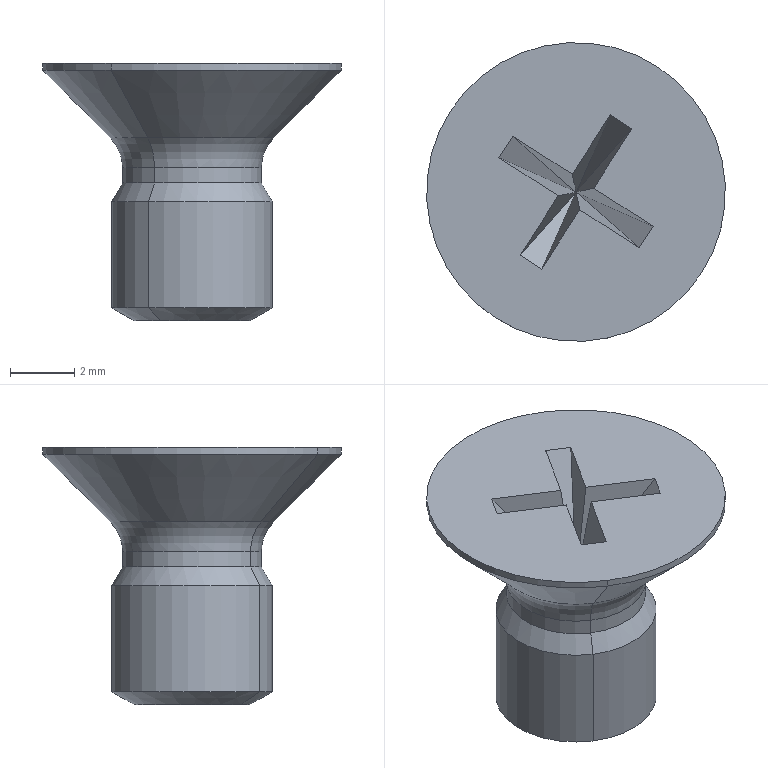Component | SolidWorks | MGL-PACK-03-00Fixture-1_PhillipsCountersunkScrewM5_8[GB_T819.1-2000]-1 | 1 solid | 28 faces | box 9.3 x 9.3 x 8 mm | volume 197 mm3 | plane 14 | cone 6 | cylinder 6 | torus 2 | commonest cylinder face diameters 5 x2 4.33 x2 9.3 x2
STEP:
#1=CARTESIAN_POINT('',(9.113,1.674,0.6496));
#2=VERTEX_POINT('',#1);
#3=CARTESIAN_POINT('',(9.036,1.554,0.6496));
#4=VERTEX_POINT('',#3);
#5=CARTESIAN_POINT('',(9.075,1.614,0.6496));
#6=DIRECTION('',(-0.,-0.,-1.));
#7=DIRECTION('',(0.5408,0.8411,0.));
#8=AXIS2_PLACEMENT_3D('',#5,#6,#7);
#9=CIRCLE('',#8,0.07115);
#10=EDGE_CURVE('',#2,#4,#9,.T.);
#11=ORIENTED_EDGE('',*,*,#10,.F.);
#12=CARTESIAN_POINT('',(9.128,1.697,0.6652));
#13=VERTEX_POINT('',#12);
#14=CARTESIAN_POINT('',(9.128,1.697,0.6652));
#15=DIRECTION('',(0.4696,0.7304,0.4959));
#16=VECTOR('',#15,39.37);
#17=LINE('',#14,#16);
#18=EDGE_CURVE('',#2,#13,#17,.T.);
#19=ORIENTED_EDGE('',*,*,#18,.T.);
#20=CARTESIAN_POINT('',(9.022,1.531,0.6652));
#21=VERTEX_POINT('',#20);
#22=CARTESIAN_POINT('',(9.075,1.614,0.6652));
#23=DIRECTION('',(-0.,-0.,-1.));
#24=DIRECTION('',(0.5408,0.8411,0.));
#25=AXIS2_PLACEMENT_3D('',#22,#23,#24);
#26=CIRCLE('',#25,0.09843);
#27=EDGE_CURVE('',#13,#21,#26,.T.);
#28=ORIENTED_EDGE('',*,*,#27,.T.);
#29=CARTESIAN_POINT('',(9.022,1.531,0.6652));
#30=DIRECTION('',(-0.4696,-0.7304,0.4959));
#31=VECTOR('',#30,39.37);
#32=LINE('',#29,#31);
#33=EDGE_CURVE('',#4,#21,#32,.T.);
#34=ORIENTED_EDGE('',*,*,#33,.F.);
#35=EDGE_LOOP('',(#11,#19,#28,#34));
#36=FACE_OUTER_BOUND('',#35,.T.);
#37=CARTESIAN_POINT('',(9.075,1.614,0.6652));
#38=DIRECTION('',(0.,0.,1.));
#39=DIRECTION('',(-0.5408,-0.8411,0.));
#40=AXIS2_PLACEMENT_3D('',#37,#38,#39);
#41=CONICAL_SURFACE('',#40,0.09843,1.052);
#42=ADVANCED_FACE('',(#36),#41,.T.);
#43=ORIENTED_EDGE('',*,*,#27,.F.);
#44=CARTESIAN_POINT('',(9.128,1.697,0.7953));
#45=VERTEX_POINT('',#44);
#46=CARTESIAN_POINT('',(9.128,1.697,0.9646));
#47=DIRECTION('',(0.,0.,1.));
#48=VECTOR('',#47,39.37);
#49=LINE('',#46,#48);
#50=EDGE_CURVE('',#13,#45,#49,.T.);
#51=ORIENTED_EDGE('',*,*,#50,.T.);
#52=CARTESIAN_POINT('',(9.022,1.531,0.7953));
#53=VERTEX_POINT('',#52);
#54=CARTESIAN_POINT('',(9.075,1.614,0.7953));
#55=DIRECTION('',(0.,0.,1.));
#56=DIRECTION('',(-0.5408,-0.8411,0.));
#57=AXIS2_PLACEMENT_3D('',#54,#55,#56);
#58=CIRCLE('',#57,0.09843);
#59=EDGE_CURVE('',#53,#45,#58,.T.);
#60=ORIENTED_EDGE('',*,*,#59,.F.);
#61=CARTESIAN_POINT('',(9.022,1.531,0.9646));
#62=DIRECTION('',(0.,0.,1.));
#63=VECTOR('',#62,39.37);
#64=LINE('',#61,#63);
#65=EDGE_CURVE('',#21,#53,#64,.T.);
#66=ORIENTED_EDGE('',*,*,#65,.F.);
#67=EDGE_LOOP('',(#43,#51,#60,#66));
#68=FACE_OUTER_BOUND('',#67,.T.);
#69=CARTESIAN_POINT('',(9.075,1.614,0.9646));
#70=DIRECTION('',(0.,0.,1.));
#71=DIRECTION('',(-0.5408,-0.8411,0.));
#72=AXIS2_PLACEMENT_3D('',#69,#70,#71);
#73=CYLINDRICAL_SURFACE('',#72,0.09843);
#74=ADVANCED_FACE('',(#68),#73,.T.);
#75=CARTESIAN_POINT('',(9.029,1.542,0.8181));
#76=VERTEX_POINT('',#75);
#77=CARTESIAN_POINT('',(9.121,1.686,0.8181));
#78=VERTEX_POINT('',#77);
#79=CARTESIAN_POINT('',(9.075,1.614,0.8181));
#80=DIRECTION('',(0.,0.,1.));
#81=DIRECTION('',(-0.5408,-0.8411,0.));
#82=AXIS2_PLACEMENT_3D('',#79,#80,#81);
#83=CIRCLE('',#82,0.08524);
#84=EDGE_CURVE('',#76,#78,#83,.T.);
#85=ORIENTED_EDGE('',*,*,#84,.F.);
#86=CARTESIAN_POINT('',(9.022,1.531,0.7953));
#87=DIRECTION('',(-0.2704,-0.4206,-0.866));
#88=VECTOR('',#87,39.37);
#89=LINE('',#86,#88);
#90=EDGE_CURVE('',#76,#53,#89,.T.);
#91=ORIENTED_EDGE('',*,*,#90,.T.);
#92=ORIENTED_EDGE('',*,*,#59,.T.);
#93=CARTESIAN_POINT('',(9.128,1.697,0.7953));
#94=DIRECTION('',(0.2704,0.4206,-0.866));
#95=VECTOR('',#94,39.37);
#96=LINE('',#93,#95);
#97=EDGE_CURVE('',#78,#45,#96,.T.);
#98=ORIENTED_EDGE('',*,*,#97,.F.);
#99=EDGE_LOOP('',(#85,#91,#92,#98));
#100=FACE_OUTER_BOUND('',#99,.T.);
#101=CARTESIAN_POINT('',(9.075,1.614,0.7953));
#102=DIRECTION('',(-0.,-0.,-1.));
#103=DIRECTION('',(0.5408,0.8411,0.));
#104=AXIS2_PLACEMENT_3D('',#101,#102,#103);
#105=CONICAL_SURFACE('',#104,0.09843,0.5236);
#106=ADVANCED_FACE('',(#100),#105,.T.);
#107=ORIENTED_EDGE('',*,*,#84,.T.);
#108=CARTESIAN_POINT('',(9.121,1.686,0.8371));
#109=VERTEX_POINT('',#108);
#110=CARTESIAN_POINT('',(9.121,1.686,0.9646));
#111=DIRECTION('',(0.,0.,1.));
#112=VECTOR('',#111,39.37);
#113=LINE('',#110,#112);
#114=EDGE_CURVE('',#78,#109,#113,.T.);
#115=ORIENTED_EDGE('',*,*,#114,.T.);
#116=CARTESIAN_POINT('',(9.029,1.542,0.8371));
#117=VERTEX_POINT('',#116);
#118=CARTESIAN_POINT('',(9.075,1.614,0.8371));
#119=DIRECTION('',(0.,0.,1.));
#120=DIRECTION('',(-0.5408,-0.8411,0.));
#121=AXIS2_PLACEMENT_3D('',#118,#119,#120);
#122=CIRCLE('',#121,0.08524);
#123=EDGE_CURVE('',#117,#109,#122,.T.);
#124=ORIENTED_EDGE('',*,*,#123,.F.);
#125=CARTESIAN_POINT('',(9.029,1.542,0.9646));
#126=DIRECTION('',(0.,0.,1.));
#127=VECTOR('',#126,39.37);
#128=LINE('',#125,#127);
#129=EDGE_CURVE('',#76,#117,#128,.T.);
#130=ORIENTED_EDGE('',*,*,#129,.F.);
#131=EDGE_LOOP('',(#107,#115,#124,#130));
#132=FACE_OUTER_BOUND('',#131,.T.);
#133=CARTESIAN_POINT('',(9.075,1.614,0.9646));
#134=DIRECTION('',(0.,0.,1.));
#135=DIRECTION('',(-0.5408,-0.8411,0.));
#136=AXIS2_PLACEMENT_3D('',#133,#134,#135);
#137=CYLINDRICAL_SURFACE('',#136,0.08524);
#138=ADVANCED_FACE('',(#132),#137,.T.);
#139=CARTESIAN_POINT('',(9.129,1.698,0.8733));
#140=VERTEX_POINT('',#139);
#141=CARTESIAN_POINT('',(9.021,1.53,0.8733));
#142=VERTEX_POINT('',#141);
#143=CARTESIAN_POINT('',(9.075,1.614,0.8733));
#144=DIRECTION('',(0.,0.,1.));
#145=DIRECTION('',(-0.5408,-0.8411,0.));
#146=AXIS2_PLACEMENT_3D('',#143,#144,#145);
#147=CIRCLE('',#146,0.1002);
#148=EDGE_CURVE('',#140,#142,#147,.T.);
#149=ORIENTED_EDGE('',*,*,#148,.F.);
#150=CARTESIAN_POINT('',(9.149,1.729,0.8371));
#151=DIRECTION('',(0.8411,-0.5408,0.));
#152=DIRECTION('',(0.5408,0.8411,0.));
#153=AXIS2_PLACEMENT_3D('',#150,#151,#152);
#154=CIRCLE('',#153,0.05118);
#155=EDGE_CURVE('',#140,#109,#154,.T.);
#156=ORIENTED_EDGE('',*,*,#155,.T.);
#157=CARTESIAN_POINT('',(9.075,1.614,0.8371));
#158=DIRECTION('',(0.,0.,1.));
#159=DIRECTION('',(-0.5408,-0.8411,0.));
#160=AXIS2_PLACEMENT_3D('',#157,#158,#159);
#161=CIRCLE('',#160,0.08524);
#162=EDGE_CURVE('',#109,#117,#161,.T.);
#163=ORIENTED_EDGE('',*,*,#162,.T.);
#164=CARTESIAN_POINT('',(9.001,1.499,0.8371));
#165=DIRECTION('',(-0.8411,0.5408,-0.));
#166=DIRECTION('',(-0.5408,-0.8411,0.));
#167=AXIS2_PLACEMENT_3D('',#164,#165,#166);
#168=CIRCLE('',#167,0.05118);
#169=EDGE_CURVE('',#142,#117,#168,.T.);
#170=ORIENTED_EDGE('',*,*,#169,.F.);
#171=EDGE_LOOP('',(#149,#156,#163,#170));
#172=FACE_OUTER_BOUND('',#171,.T.);
#173=CARTESIAN_POINT('',(9.075,1.614,0.8371));
#174=DIRECTION('',(0.,0.,1.));
#175=DIRECTION('',(-0.5408,-0.8411,0.));
#176=AXIS2_PLACEMENT_3D('',#173,#174,#175);
#177=TOROIDAL_SURFACE('',#176,0.1364,0.05118);
#178=ADVANCED_FACE('',(#172),#177,.F.);
#179=CARTESIAN_POINT('',(9.075,1.614,0.8733));
#180=DIRECTION('',(0.,0.,1.));
#181=DIRECTION('',(-0.5408,-0.8411,0.));
#182=AXIS2_PLACEMENT_3D('',#179,#180,#181);
#183=CIRCLE('',#182,0.1002);
#184=EDGE_CURVE('',#142,#140,#183,.T.);
#185=ORIENTED_EDGE('',*,*,#184,.T.);
#186=CARTESIAN_POINT('',(9.174,1.768,0.9561));
#187=VERTEX_POINT('',#186);
#188=CARTESIAN_POINT('',(9.129,1.698,0.8733));
#189=DIRECTION('',(0.3824,0.5948,0.7071));
#190=VECTOR('',#189,39.37);
#191=LINE('',#188,#190);
#192=EDGE_CURVE('',#140,#187,#191,.T.);
#193=ORIENTED_EDGE('',*,*,#192,.T.);
#194=CARTESIAN_POINT('',(8.976,1.46,0.9561));
#195=VERTEX_POINT('',#194);
#196=CARTESIAN_POINT('',(9.075,1.614,0.9561));
#197=DIRECTION('',(0.,0.,1.));
#198=DIRECTION('',(-0.5408,-0.8411,0.));
#199=AXIS2_PLACEMENT_3D('',#196,#197,#198);
#200=CIRCLE('',#199,0.1831);
#201=EDGE_CURVE('',#195,#187,#200,.T.);
#202=ORIENTED_EDGE('',*,*,#201,.F.);
#203=CARTESIAN_POINT('',(9.021,1.53,0.8733));
#204=DIRECTION('',(-0.3824,-0.5948,0.7071));
#205=VECTOR('',#204,39.37);
#206=LINE('',#203,#205);
#207=EDGE_CURVE('',#142,#195,#206,.T.);
#208=ORIENTED_EDGE('',*,*,#207,.F.);
#209=EDGE_LOOP('',(#185,#193,#202,#208));
#210=FACE_OUTER_BOUND('',#209,.T.);
#211=CARTESIAN_POINT('',(9.075,1.614,0.8733));
#212=DIRECTION('',(0.,0.,1.));
#213=DIRECTION('',(-0.5408,-0.8411,0.));
#214=AXIS2_PLACEMENT_3D('',#211,#212,#213);
#215=CONICAL_SURFACE('',#214,0.1002,0.7854);
#216=ADVANCED_FACE('',(#210),#215,.T.);
#217=ORIENTED_EDGE('',*,*,#201,.T.);
#218=CARTESIAN_POINT('',(9.174,1.768,0.9646));
#219=VERTEX_POINT('',#218);
#220=CARTESIAN_POINT('',(9.174,1.768,0.9646));
#221=DIRECTION('',(0.,0.,1.));
#222=VECTOR('',#221,39.37);
#223=LINE('',#220,#222);
#224=EDGE_CURVE('',#187,#219,#223,.T.);
#225=ORIENTED_EDGE('',*,*,#224,.T.);
#226=CARTESIAN_POINT('',(8.976,1.46,0.9646));
#227=VERTEX_POINT('',#226);
#228=CARTESIAN_POINT('',(9.075,1.614,0.9646));
#229=DIRECTION('',(0.,0.,1.));
#230=DIRECTION('',(-0.5408,-0.8411,0.));
#231=AXIS2_PLACEMENT_3D('',#228,#229,#230);
#232=CIRCLE('',#231,0.1831);
#233=EDGE_CURVE('',#227,#219,#232,.T.);
#234=ORIENTED_EDGE('',*,*,#233,.F.);
#235=CARTESIAN_POINT('',(8.976,1.46,0.9646));
#236=DIRECTION('',(0.,0.,1.));
#237=VECTOR('',#236,39.37);
#238=LINE('',#235,#237);
#239=EDGE_CURVE('',#195,#227,#238,.T.);
#240=ORIENTED_EDGE('',*,*,#239,.F.);
#241=EDGE_LOOP('',(#217,#225,#234,#240));
#242=FACE_OUTER_BOUND('',#241,.T.);
#243=CARTESIAN_POINT('',(9.075,1.614,0.9646));
#244=DIRECTION('',(0.,0.,1.));
#245=DIRECTION('',(-0.5408,-0.8411,0.));
#246=AXIS2_PLACEMENT_3D('',#243,#244,#245);
#247=CYLINDRICAL_SURFACE('',#246,0.1831);
#248=ADVANCED_FACE('',(#242),#247,.T.);
#249=ORIENTED_EDGE('',*,*,#233,.T.);
#250=CARTESIAN_POINT('',(9.075,1.614,0.9646));
#251=DIRECTION('',(0.,0.,1.));
#252=DIRECTION('',(-0.5408,-0.8411,0.));
#253=AXIS2_PLACEMENT_3D('',#250,#251,#252);
#254=CIRCLE('',#253,0.1831);
#255=EDGE_CURVE('',#219,#227,#254,.T.);
#256=ORIENTED_EDGE('',*,*,#255,.T.);
#257=EDGE_LOOP('',(#249,#256));
#258=FACE_OUTER_BOUND('',#257,.T.);
#259=CARTESIAN_POINT('',(9.08,1.592,0.9646));
#260=VERTEX_POINT('',#259);
#261=CARTESIAN_POINT('',(9.152,1.546,0.9646));
#262=VERTEX_POINT('',#261);
#263=CARTESIAN_POINT('',(9.152,1.546,0.9646));
#264=DIRECTION('',(0.8411,-0.5408,0.));
#265=VECTOR('',#264,39.37);
#266=LINE('',#263,#265);
#267=EDGE_CURVE('',#260,#262,#266,.T.);
#268=ORIENTED_EDGE('',*,*,#267,.F.);
#269=CARTESIAN_POINT('',(9.033,1.52,0.9646));
#270=VERTEX_POINT('',#269);
#271=CARTESIAN_POINT('',(9.143,1.692,0.9646));
#272=DIRECTION('',(0.5408,0.8411,-0.));
#273=VECTOR('',#272,39.37);
#274=LINE('',#271,#273);
#275=EDGE_CURVE('',#270,#260,#274,.T.);
#276=ORIENTED_EDGE('',*,*,#275,.F.);
#277=CARTESIAN_POINT('',(9.006,1.537,0.9646));
#278=VERTEX_POINT('',#277);
#279=CARTESIAN_POINT('',(9.033,1.52,0.9646));
#280=DIRECTION('',(0.8411,-0.5408,0.));
#281=VECTOR('',#280,39.37);
#282=LINE('',#279,#281);
#283=EDGE_CURVE('',#278,#270,#282,.T.);
#284=ORIENTED_EDGE('',*,*,#283,.F.);
#285=CARTESIAN_POINT('',(9.053,1.609,0.9646));
#286=VERTEX_POINT('',#285);
#287=CARTESIAN_POINT('',(9.117,1.709,0.9646));
#288=DIRECTION('',(-0.5408,-0.8411,0.));
#289=VECTOR('',#288,39.37);
#290=LINE('',#287,#289);
#291=EDGE_CURVE('',#286,#278,#290,.T.);
#292=ORIENTED_EDGE('',*,*,#291,.F.);
#293=CARTESIAN_POINT('',(8.98,1.656,0.9646));
#294=VERTEX_POINT('',#293);
#295=CARTESIAN_POINT('',(9.152,1.546,0.9646));
#296=DIRECTION('',(0.8411,-0.5408,0.));
#297=VECTOR('',#296,39.37);
#298=LINE('',#295,#297);
#299=EDGE_CURVE('',#294,#286,#298,.T.);
#300=ORIENTED_EDGE('',*,*,#299,.F.);
#301=CARTESIAN_POINT('',(8.997,1.683,0.9646));
#302=VERTEX_POINT('',#301);
#303=CARTESIAN_POINT('',(8.98,1.656,0.9646));
#304=DIRECTION('',(-0.5408,-0.8411,0.));
#305=VECTOR('',#304,39.37);
#306=LINE('',#303,#305);
#307=EDGE_CURVE('',#302,#294,#306,.T.);
#308=ORIENTED_EDGE('',*,*,#307,.F.);
#309=CARTESIAN_POINT('',(9.07,1.636,0.9646));
#310=VERTEX_POINT('',#309);
#311=CARTESIAN_POINT('',(9.169,1.572,0.9646));
#312=DIRECTION('',(-0.8411,0.5408,-0.));
#313=VECTOR('',#312,39.37);
#314=LINE('',#311,#313);
#315=EDGE_CURVE('',#310,#302,#314,.T.);
#316=ORIENTED_EDGE('',*,*,#315,.F.);
#317=CARTESIAN_POINT('',(9.117,1.709,0.9646));
#318=VERTEX_POINT('',#317);
#319=CARTESIAN_POINT('',(9.117,1.709,0.9646));
#320=DIRECTION('',(-0.5408,-0.8411,0.));
#321=VECTOR('',#320,39.37);
#322=LINE('',#319,#321);
#323=EDGE_CURVE('',#318,#310,#322,.T.);
#324=ORIENTED_EDGE('',*,*,#323,.F.);
#325=CARTESIAN_POINT('',(9.143,1.692,0.9646));
#326=VERTEX_POINT('',#325);
#327=CARTESIAN_POINT('',(9.143,1.692,0.9646));
#328=DIRECTION('',(-0.8411,0.5408,-0.));
#329=VECTOR('',#328,39.37);
#330=LINE('',#327,#329);
#331=EDGE_CURVE('',#326,#318,#330,.T.);
#332=ORIENTED_EDGE('',*,*,#331,.F.);
#333=CARTESIAN_POINT('',(9.097,1.619,0.9646));
#334=VERTEX_POINT('',#333);
#335=CARTESIAN_POINT('',(9.143,1.692,0.9646));
#336=DIRECTION('',(0.5408,0.8411,-0.));
#337=VECTOR('',#336,39.37);
#338=LINE('',#335,#337);
#339=EDGE_CURVE('',#334,#326,#338,.T.);
#340=ORIENTED_EDGE('',*,*,#339,.F.);
#341=CARTESIAN_POINT('',(9.169,1.572,0.9646));
#342=VERTEX_POINT('',#341);
#343=CARTESIAN_POINT('',(9.169,1.572,0.9646));
#344=DIRECTION('',(-0.8411,0.5408,-0.));
#345=VECTOR('',#344,39.37);
#346=LINE('',#343,#345);
#347=EDGE_CURVE('',#342,#334,#346,.T.);
#348=ORIENTED_EDGE('',*,*,#347,.F.);
#349=CARTESIAN_POINT('',(9.152,1.546,0.9646));
#350=DIRECTION('',(0.5408,0.8411,-0.));
#351=VECTOR('',#350,39.37);
#352=LINE('',#349,#351);
#353=EDGE_CURVE('',#262,#342,#352,.T.);
#354=ORIENTED_EDGE('',*,*,#353,.F.);
#355=EDGE_LOOP('',(#268,#276,#284,#292,#300,#308,#316,#324,#332,#340,#348,#354));
#356=FACE_BOUND('',#355,.T.);
#357=CARTESIAN_POINT('',(9.075,1.614,0.9646));
#358=DIRECTION('',(-0.,-0.,-1.));
#359=DIRECTION('',(0.5408,0.8411,-0.));
#360=AXIS2_PLACEMENT_3D('',#357,#358,#359);
#361=PLANE('',#360);
#362=ADVANCED_FACE('',(#258,#356),#361,.F.);
#363=ORIENTED_EDGE('',*,*,#275,.T.);
#364=CARTESIAN_POINT('',(9.075,1.614,0.8386));
#365=VERTEX_POINT('',#364);
#366=CARTESIAN_POINT('',(9.075,1.614,0.8386));
#367=DIRECTION('',(-0.03697,0.1701,-0.9847));
#368=VECTOR('',#367,39.37);
#369=LINE('',#366,#368);
#370=EDGE_CURVE('',#260,#365,#369,.T.);
#371=ORIENTED_EDGE('',*,*,#370,.T.);
#372=CARTESIAN_POINT('',(9.033,1.52,0.9646));
#373=DIRECTION('',(0.2582,0.5802,-0.7725));
#374=VECTOR('',#373,39.37);
#375=LINE('',#372,#374);
#376=EDGE_CURVE('',#270,#365,#375,.T.);
#377=ORIENTED_EDGE('',*,*,#376,.F.);
#378=EDGE_LOOP('',(#363,#371,#377));
#379=FACE_OUTER_BOUND('',#378,.T.);
#380=CARTESIAN_POINT('',(9.075,1.614,0.8386));
#381=DIRECTION('',(-0.8347,0.5366,0.124));
#382=DIRECTION('',(-0.1043,0.06708,-0.9923));
#383=AXIS2_PLACEMENT_3D('',#380,#381,#382);
#384=PLANE('',#383);
#385=ADVANCED_FACE('',(#379),#384,.T.);
#386=CARTESIAN_POINT('',(9.143,1.692,0.9646));
#387=DIRECTION('',(-0.4207,-0.4757,-0.7725));
#388=VECTOR('',#387,39.37);
#389=LINE('',#386,#388);
#390=EDGE_CURVE('',#326,#365,#389,.T.);
#391=ORIENTED_EDGE('',*,*,#390,.T.);
#392=CARTESIAN_POINT('',(9.075,1.614,0.8386));
#393=DIRECTION('',(0.1701,0.03697,0.9847));
#394=VECTOR('',#393,39.37);
#395=LINE('',#392,#394);
#396=EDGE_CURVE('',#365,#334,#395,.T.);
#397=ORIENTED_EDGE('',*,*,#396,.T.);
#398=ORIENTED_EDGE('',*,*,#339,.T.);
#399=EDGE_LOOP('',(#391,#397,#398));
#400=FACE_OUTER_BOUND('',#399,.T.);
#401=CARTESIAN_POINT('',(9.075,1.614,0.8386));
#402=DIRECTION('',(-0.8347,0.5366,0.124));
#403=DIRECTION('',(-0.1043,0.06708,-0.9923));
#404=AXIS2_PLACEMENT_3D('',#401,#402,#403);
#405=PLANE('',#404);
#406=ADVANCED_FACE('',(#400),#405,.T.);
#407=CARTESIAN_POINT('',(9.006,1.537,0.9646));
#408=DIRECTION('',(0.4207,0.4757,-0.7725));
#409=VECTOR('',#408,39.37);
#410=LINE('',#407,#409);
#411=EDGE_CURVE('',#278,#365,#410,.T.);
#412=ORIENTED_EDGE('',*,*,#411,.T.);
#413=CARTESIAN_POINT('',(9.075,1.614,0.8386));
#414=DIRECTION('',(-0.1701,-0.03697,0.9847));
#415=VECTOR('',#414,39.37);
#416=LINE('',#413,#415);
#417=EDGE_CURVE('',#365,#286,#416,.T.);
#418=ORIENTED_EDGE('',*,*,#417,.T.);
#419=ORIENTED_EDGE('',*,*,#291,.T.);
#420=EDGE_LOOP('',(#412,#418,#419));
#421=FACE_OUTER_BOUND('',#420,.T.);
#422=CARTESIAN_POINT('',(9.075,1.614,0.8386));
#423=DIRECTION('',(0.8347,-0.5366,0.124));
#424=DIRECTION('',(-0.1043,0.06708,0.9923));
#425=AXIS2_PLACEMENT_3D('',#422,#423,#424);
#426=PLANE('',#425);
#427=ADVANCED_FACE('',(#421),#426,.T.);
#428=ORIENTED_EDGE('',*,*,#323,.T.);
#429=CARTESIAN_POINT('',(9.075,1.614,0.8386));
#430=DIRECTION('',(0.03697,-0.1701,-0.9847));
#431=VECTOR('',#430,39.37);
#432=LINE('',#429,#431);
#433=EDGE_CURVE('',#310,#365,#432,.T.);
#434=ORIENTED_EDGE('',*,*,#433,.T.);
#435=CARTESIAN_POINT('',(9.117,1.709,0.9646));
#436=DIRECTION('',(-0.2582,-0.5802,-0.7725));
#437=VECTOR('',#436,39.37);
#438=LINE('',#435,#437);
#439=EDGE_CURVE('',#318,#365,#438,.T.);
#440=ORIENTED_EDGE('',*,*,#439,.F.);
#441=EDGE_LOOP('',(#428,#434,#440));
#442=FACE_OUTER_BOUND('',#441,.T.);
#443=CARTESIAN_POINT('',(9.075,1.614,0.8386));
#444=DIRECTION('',(0.8347,-0.5366,0.124));
#445=DIRECTION('',(-0.1043,0.06708,0.9923));
#446=AXIS2_PLACEMENT_3D('',#443,#444,#445);
#447=PLANE('',#446);
#448=ADVANCED_FACE('',(#442),#447,.T.);
#449=ORIENTED_EDGE('',*,*,#224,.F.);
#450=CARTESIAN_POINT('',(9.075,1.614,0.9561));
#451=DIRECTION('',(0.,0.,1.));
#452=DIRECTION('',(-0.5408,-0.8411,0.));
#453=AXIS2_PLACEMENT_3D('',#450,#451,#452);
#454=CIRCLE('',#453,0.1831);
#455=EDGE_CURVE('',#187,#195,#454,.T.);
#456=ORIENTED_EDGE('',*,*,#455,.T.);
#457=ORIENTED_EDGE('',*,*,#239,.T.);
#458=ORIENTED_EDGE('',*,*,#255,.F.);
#459=EDGE_LOOP('',(#449,#456,#457,#458));
#460=FACE_OUTER_BOUND('',#459,.T.);
#461=CARTESIAN_POINT('',(9.075,1.614,0.9646));
#462=DIRECTION('',(0.,0.,1.));
#463=DIRECTION('',(-0.5408,-0.8411,0.));
#464=AXIS2_PLACEMENT_3D('',#461,#462,#463);
#465=CYLINDRICAL_SURFACE('',#464,0.1831);
#466=ADVANCED_FACE('',(#460),#465,.T.);
#467=ORIENTED_EDGE('',*,*,#192,.F.);
#468=ORIENTED_EDGE('',*,*,#148,.T.);
#469=ORIENTED_EDGE('',*,*,#207,.T.);
#470=ORIENTED_EDGE('',*,*,#455,.F.);
#471=EDGE_LOOP('',(#467,#468,#469,#470));
#472=FACE_OUTER_BOUND('',#471,.T.);
#473=CARTESIAN_POINT('',(9.075,1.614,0.8733));
#474=DIRECTION('',(0.,0.,1.));
#475=DIRECTION('',(-0.5408,-0.8411,0.));
#476=AXIS2_PLACEMENT_3D('',#473,#474,#475);
#477=CONICAL_SURFACE('',#476,0.1002,0.7854);
#478=ADVANCED_FACE('',(#472),#477,.T.);
#479=ORIENTED_EDGE('',*,*,#155,.F.);
#480=ORIENTED_EDGE('',*,*,#184,.F.);
#481=ORIENTED_EDGE('',*,*,#169,.T.);
#482=ORIENTED_EDGE('',*,*,#123,.T.);
#483=EDGE_LOOP('',(#479,#480,#481,#482));
#484=FACE_OUTER_BOUND('',#483,.T.);
#485=CARTESIAN_POINT('',(9.075,1.614,0.8371));
#486=DIRECTION('',(0.,0.,1.));
#487=DIRECTION('',(-0.5408,-0.8411,0.));
#488=AXIS2_PLACEMENT_3D('',#485,#486,#487);
#489=TOROIDAL_SURFACE('',#488,0.1364,0.05118);
#490=ADVANCED_FACE('',(#484),#489,.F.);
#491=ORIENTED_EDGE('',*,*,#114,.F.);
#492=CARTESIAN_POINT('',(9.075,1.614,0.8181));
#493=DIRECTION('',(0.,0.,1.));
#494=DIRECTION('',(-0.5408,-0.8411,0.));
#495=AXIS2_PLACEMENT_3D('',#492,#493,#494);
#496=CIRCLE('',#495,0.08524);
#497=EDGE_CURVE('',#78,#76,#496,.T.);
#498=ORIENTED_EDGE('',*,*,#497,.T.);
#499=ORIENTED_EDGE('',*,*,#129,.T.);
#500=ORIENTED_EDGE('',*,*,#162,.F.);
#501=EDGE_LOOP('',(#491,#498,#499,#500));
#502=FACE_OUTER_BOUND('',#501,.T.);
#503=CARTESIAN_POINT('',(9.075,1.614,0.9646));
#504=DIRECTION('',(0.,0.,1.));
#505=DIRECTION('',(-0.5408,-0.8411,0.));
#506=AXIS2_PLACEMENT_3D('',#503,#504,#505);
#507=CYLINDRICAL_SURFACE('',#506,0.08524);
#508=ADVANCED_FACE('',(#502),#507,.T.);
#509=ORIENTED_EDGE('',*,*,#90,.F.);
#510=ORIENTED_EDGE('',*,*,#497,.F.);
#511=ORIENTED_EDGE('',*,*,#97,.T.);
#512=CARTESIAN_POINT('',(9.075,1.614,0.7953));
#513=DIRECTION('',(0.,0.,1.));
#514=DIRECTION('',(-0.5408,-0.8411,0.));
#515=AXIS2_PLACEMENT_3D('',#512,#513,#514);
#516=CIRCLE('',#515,0.09843);
#517=EDGE_CURVE('',#45,#53,#516,.T.);
#518=ORIENTED_EDGE('',*,*,#517,.T.);
#519=EDGE_LOOP('',(#509,#510,#511,#518));
#520=FACE_OUTER_BOUND('',#519,.T.);
#521=CARTESIAN_POINT('',(9.075,1.614,0.7953));
#522=DIRECTION('',(-0.,-0.,-1.));
#523=DIRECTION('',(0.5408,0.8411,0.));
#524=AXIS2_PLACEMENT_3D('',#521,#522,#523);
#525=CONICAL_SURFACE('',#524,0.09843,0.5236);
#526=ADVANCED_FACE('',(#520),#525,.T.);
#527=ORIENTED_EDGE('',*,*,#50,.F.);
#528=CARTESIAN_POINT('',(9.075,1.614,0.6652));
#529=DIRECTION('',(-0.,-0.,-1.));
#530=DIRECTION('',(0.5408,0.8411,0.));
#531=AXIS2_PLACEMENT_3D('',#528,#529,#530);
#532=CIRCLE('',#531,0.09843);
#533=EDGE_CURVE('',#21,#13,#532,.T.);
#534=ORIENTED_EDGE('',*,*,#533,.F.);
#535=ORIENTED_EDGE('',*,*,#65,.T.);
#536=ORIENTED_EDGE('',*,*,#517,.F.);
#537=EDGE_LOOP('',(#527,#534,#535,#536));
#538=FACE_OUTER_BOUND('',#537,.T.);
#539=CARTESIAN_POINT('',(9.075,1.614,0.9646));
#540=DIRECTION('',(0.,0.,1.));
#541=DIRECTION('',(-0.5408,-0.8411,0.));
#542=AXIS2_PLACEMENT_3D('',#539,#540,#541);
#543=CYLINDRICAL_SURFACE('',#542,0.09843);
#544=ADVANCED_FACE('',(#538),#543,.T.);
#545=ORIENTED_EDGE('',*,*,#18,.F.);
#546=CARTESIAN_POINT('',(9.075,1.614,0.6496));
#547=DIRECTION('',(-0.,-0.,-1.));
#548=DIRECTION('',(0.5408,0.8411,0.));
#549=AXIS2_PLACEMENT_3D('',#546,#547,#548);
#550=CIRCLE('',#549,0.07115);
#551=EDGE_CURVE('',#4,#2,#550,.T.);
#552=ORIENTED_EDGE('',*,*,#551,.F.);
#553=ORIENTED_EDGE('',*,*,#33,.T.);
#554=ORIENTED_EDGE('',*,*,#533,.T.);
#555=EDGE_LOOP('',(#545,#552,#553,#554));
#556=FACE_OUTER_BOUND('',#555,.T.);
#557=CARTESIAN_POINT('',(9.075,1.614,0.6652));
#558=DIRECTION('',(0.,0.,1.));
#559=DIRECTION('',(-0.5408,-0.8411,0.));
#560=AXIS2_PLACEMENT_3D('',#557,#558,#559);
#561=CONICAL_SURFACE('',#560,0.09843,1.052);
#562=ADVANCED_FACE('',(#556),#561,.T.);
#563=ORIENTED_EDGE('',*,*,#551,.T.);
#564=ORIENTED_EDGE('',*,*,#10,.T.);
#565=EDGE_LOOP('',(#563,#564));
#566=FACE_OUTER_BOUND('',#565,.T.);
#567=CARTESIAN_POINT('',(9.158,1.561,0.6496));
#568=DIRECTION('',(0.,0.,1.));
#569=DIRECTION('',(-0.5408,-0.8411,0.));
#570=AXIS2_PLACEMENT_3D('',#567,#568,#569);
#571=PLANE('',#570);
#572=ADVANCED_FACE('',(#566),#571,.F.);
#573=ORIENTED_EDGE('',*,*,#390,.F.);
#574=ORIENTED_EDGE('',*,*,#331,.T.);
#575=ORIENTED_EDGE('',*,*,#439,.T.);
#576=EDGE_LOOP('',(#573,#574,#575));
#577=FACE_OUTER_BOUND('',#576,.T.);
#578=CARTESIAN_POINT('',(9.143,1.692,0.9646));
#579=DIRECTION('',(0.4197,0.6528,-0.6306));
#580=DIRECTION('',(0.341,0.5304,0.7761));
#581=AXIS2_PLACEMENT_3D('',#578,#579,#580);
#582=PLANE('',#581);
#583=ADVANCED_FACE('',(#577),#582,.F.);
#584=ORIENTED_EDGE('',*,*,#411,.F.);
#585=ORIENTED_EDGE('',*,*,#283,.T.);
#586=ORIENTED_EDGE('',*,*,#376,.T.);
#587=EDGE_LOOP('',(#584,#585,#586));
#588=FACE_OUTER_BOUND('',#587,.T.);
#589=CARTESIAN_POINT('',(9.006,1.537,0.9646));
#590=DIRECTION('',(-0.4197,-0.6528,-0.6306));
#591=DIRECTION('',(0.341,0.5304,-0.7761));
#592=AXIS2_PLACEMENT_3D('',#589,#590,#591);
#593=PLANE('',#592);
#594=ADVANCED_FACE('',(#588),#593,.F.);
#595=CARTESIAN_POINT('',(8.98,1.656,0.9646));
#596=DIRECTION('',(0.5802,-0.2582,-0.7725));
#597=VECTOR('',#596,39.37);
#598=LINE('',#595,#597);
#599=EDGE_CURVE('',#294,#365,#598,.T.);
#600=ORIENTED_EDGE('',*,*,#599,.F.);
#601=ORIENTED_EDGE('',*,*,#299,.T.);
#602=ORIENTED_EDGE('',*,*,#417,.F.);
#603=EDGE_LOOP('',(#600,#601,#602));
#604=FACE_OUTER_BOUND('',#603,.T.);
#605=CARTESIAN_POINT('',(9.075,1.614,0.8386));
#606=DIRECTION('',(0.5366,0.8347,0.124));
#607=DIRECTION('',(0.06708,0.1043,-0.9923));
#608=AXIS2_PLACEMENT_3D('',#605,#606,#607);
#609=PLANE('',#608);
#610=ADVANCED_FACE('',(#604),#609,.T.);
#611=ORIENTED_EDGE('',*,*,#315,.T.);
#612=CARTESIAN_POINT('',(8.997,1.683,0.9646));
#613=DIRECTION('',(0.4757,-0.4207,-0.7725));
#614=VECTOR('',#613,39.37);
#615=LINE('',#612,#614);
#616=EDGE_CURVE('',#302,#365,#615,.T.);
#617=ORIENTED_EDGE('',*,*,#616,.T.);
#618=ORIENTED_EDGE('',*,*,#433,.F.);
#619=EDGE_LOOP('',(#611,#617,#618));
#620=FACE_OUTER_BOUND('',#619,.T.);
#621=CARTESIAN_POINT('',(9.075,1.614,0.8386));
#622=DIRECTION('',(-0.5366,-0.8347,0.124));
#623=DIRECTION('',(0.06708,0.1043,0.9923));
#624=AXIS2_PLACEMENT_3D('',#621,#622,#623);
#625=PLANE('',#624);
#626=ADVANCED_FACE('',(#620),#625,.T.);
#627=ORIENTED_EDGE('',*,*,#616,.F.);
#628=ORIENTED_EDGE('',*,*,#307,.T.);
#629=ORIENTED_EDGE('',*,*,#599,.T.);
#630=EDGE_LOOP('',(#627,#628,#629));
#631=FACE_OUTER_BOUND('',#630,.T.);
#632=CARTESIAN_POINT('',(8.997,1.683,0.9646));
#633=DIRECTION('',(-0.6528,0.4197,-0.6306));
#634=DIRECTION('',(0.5304,-0.341,-0.7761));
#635=AXIS2_PLACEMENT_3D('',#632,#633,#634);
#636=PLANE('',#635);
#637=ADVANCED_FACE('',(#631),#636,.F.);
#638=ORIENTED_EDGE('',*,*,#267,.T.);
#639=CARTESIAN_POINT('',(9.152,1.546,0.9646));
#640=DIRECTION('',(-0.4757,0.4207,-0.7725));
#641=VECTOR('',#640,39.37);
#642=LINE('',#639,#641);
#643=EDGE_CURVE('',#262,#365,#642,.T.);
#644=ORIENTED_EDGE('',*,*,#643,.T.);
#645=ORIENTED_EDGE('',*,*,#370,.F.);
#646=EDGE_LOOP('',(#638,#644,#645));
#647=FACE_OUTER_BOUND('',#646,.T.);
#648=CARTESIAN_POINT('',(9.075,1.614,0.8386));
#649=DIRECTION('',(0.5366,0.8347,0.124));
#650=DIRECTION('',(0.06708,0.1043,-0.9923));
#651=AXIS2_PLACEMENT_3D('',#648,#649,#650);
#652=PLANE('',#651);
#653=ADVANCED_FACE('',(#647),#652,.T.);
#654=CARTESIAN_POINT('',(9.169,1.572,0.9646));
#655=DIRECTION('',(-0.5802,0.2582,-0.7725));
#656=VECTOR('',#655,39.37);
#657=LINE('',#654,#656);
#658=EDGE_CURVE('',#342,#365,#657,.T.);
#659=ORIENTED_EDGE('',*,*,#658,.F.);
#660=ORIENTED_EDGE('',*,*,#347,.T.);
#661=ORIENTED_EDGE('',*,*,#396,.F.);
#662=EDGE_LOOP('',(#659,#660,#661));
#663=FACE_OUTER_BOUND('',#662,.T.);
#664=CARTESIAN_POINT('',(9.075,1.614,0.8386));
#665=DIRECTION('',(-0.5366,-0.8347,0.124));
#666=DIRECTION('',(0.06708,0.1043,0.9923));
#667=AXIS2_PLACEMENT_3D('',#664,#665,#666);
#668=PLANE('',#667);
#669=ADVANCED_FACE('',(#663),#668,.T.);
#670=ORIENTED_EDGE('',*,*,#643,.F.);
#671=ORIENTED_EDGE('',*,*,#353,.T.);
#672=ORIENTED_EDGE('',*,*,#658,.T.);
#673=EDGE_LOOP('',(#670,#671,#672));
#674=FACE_OUTER_BOUND('',#673,.T.);
#675=CARTESIAN_POINT('',(9.152,1.546,0.9646));
#676=DIRECTION('',(0.6528,-0.4197,-0.6306));
#677=DIRECTION('',(0.5304,-0.341,0.7761));
#678=AXIS2_PLACEMENT_3D('',#675,#676,#677);
#679=PLANE('',#678);
#680=ADVANCED_FACE('',(#674),#679,.F.);
#681=CLOSED_SHELL('',(#42,#74,#106,#138,#178,#216,#248,#362,#385,#406,#427,#448,#466,#478,#490,#508,#526,#544,#562,#572,#583,#594,#610,#626,#637,#653,#669,#680));
#682=MANIFOLD_SOLID_BREP('',#681);
#683=CARTESIAN_POINT('',(0.,0.,0.));
#684=DIRECTION('',(0.,0.,1.));
#685=DIRECTION('',(1.,0.,0.));
#686=AXIS2_PLACEMENT_3D('',#683,#684,#685);
#687=(LENGTH_UNIT()NAMED_UNIT(*)SI_UNIT($,.METRE.));
#688=LENGTH_MEASURE_WITH_UNIT(LENGTH_MEASURE(0.0254),#687);
#689=DIMENSIONAL_EXPONENTS(1.,0.,0.,0.,0.,0.,0.);
#690=(CONVERSION_BASED_UNIT('',#688)LENGTH_UNIT()NAMED_UNIT(#689));
#691=UNCERTAINTY_MEASURE_WITH_UNIT(LENGTH_MEASURE(0.00001),#690,'','');
#692=(NAMED_UNIT(*)PLANE_ANGLE_UNIT()SI_UNIT($,.RADIAN.));
#693=(NAMED_UNIT(*)SI_UNIT($,.STERADIAN.)SOLID_ANGLE_UNIT());
#694=(GEOMETRIC_REPRESENTATION_CONTEXT(3)GLOBAL_UNCERTAINTY_ASSIGNED_CONTEXT((#691))GLOBAL_UNIT_ASSIGNED_CONTEXT((#690,#692,#693))REPRESENTATION_CONTEXT('',''));
#695=ADVANCED_BREP_SHAPE_REPRESENTATION('',(#682,#686),#694);
#696=COLOUR_RGB('',0.7922,0.8196,0.9333);
#697=FILL_AREA_STYLE_COLOUR('',#696);
#698=FILL_AREA_STYLE('',(#697));
#699=SURFACE_STYLE_FILL_AREA(#698);
#700=SURFACE_SIDE_STYLE('',(#699));
#701=SURFACE_STYLE_USAGE(.BOTH.,#700);
#702=PRESENTATION_STYLE_ASSIGNMENT((#701));
#703=STYLED_ITEM('',(#702),#682);
#704=PRESENTATION_LAYER_ASSIGNMENT('','',(#703));
#705=(LENGTH_UNIT()NAMED_UNIT(*)SI_UNIT($,.METRE.));
#706=LENGTH_MEASURE_WITH_UNIT(LENGTH_MEASURE(0.0254),#705);
#707=DIMENSIONAL_EXPONENTS(1.,0.,0.,0.,0.,0.,0.);
#708=(CONVERSION_BASED_UNIT('',#706)LENGTH_UNIT()NAMED_UNIT(#707));
#709=UNCERTAINTY_MEASURE_WITH_UNIT(LENGTH_MEASURE(0.00001),#708,'','');
#710=(NAMED_UNIT(*)PLANE_ANGLE_UNIT()SI_UNIT($,.RADIAN.));
#711=(NAMED_UNIT(*)SI_UNIT($,.STERADIAN.)SOLID_ANGLE_UNIT());
#712=(GEOMETRIC_REPRESENTATION_CONTEXT(3)GLOBAL_UNCERTAINTY_ASSIGNED_CONTEXT((#709))GLOBAL_UNIT_ASSIGNED_CONTEXT((#708,#710,#711))REPRESENTATION_CONTEXT('',''));
#713=MECHANICAL_DESIGN_GEOMETRIC_PRESENTATION_REPRESENTATION('',(#703),#712);